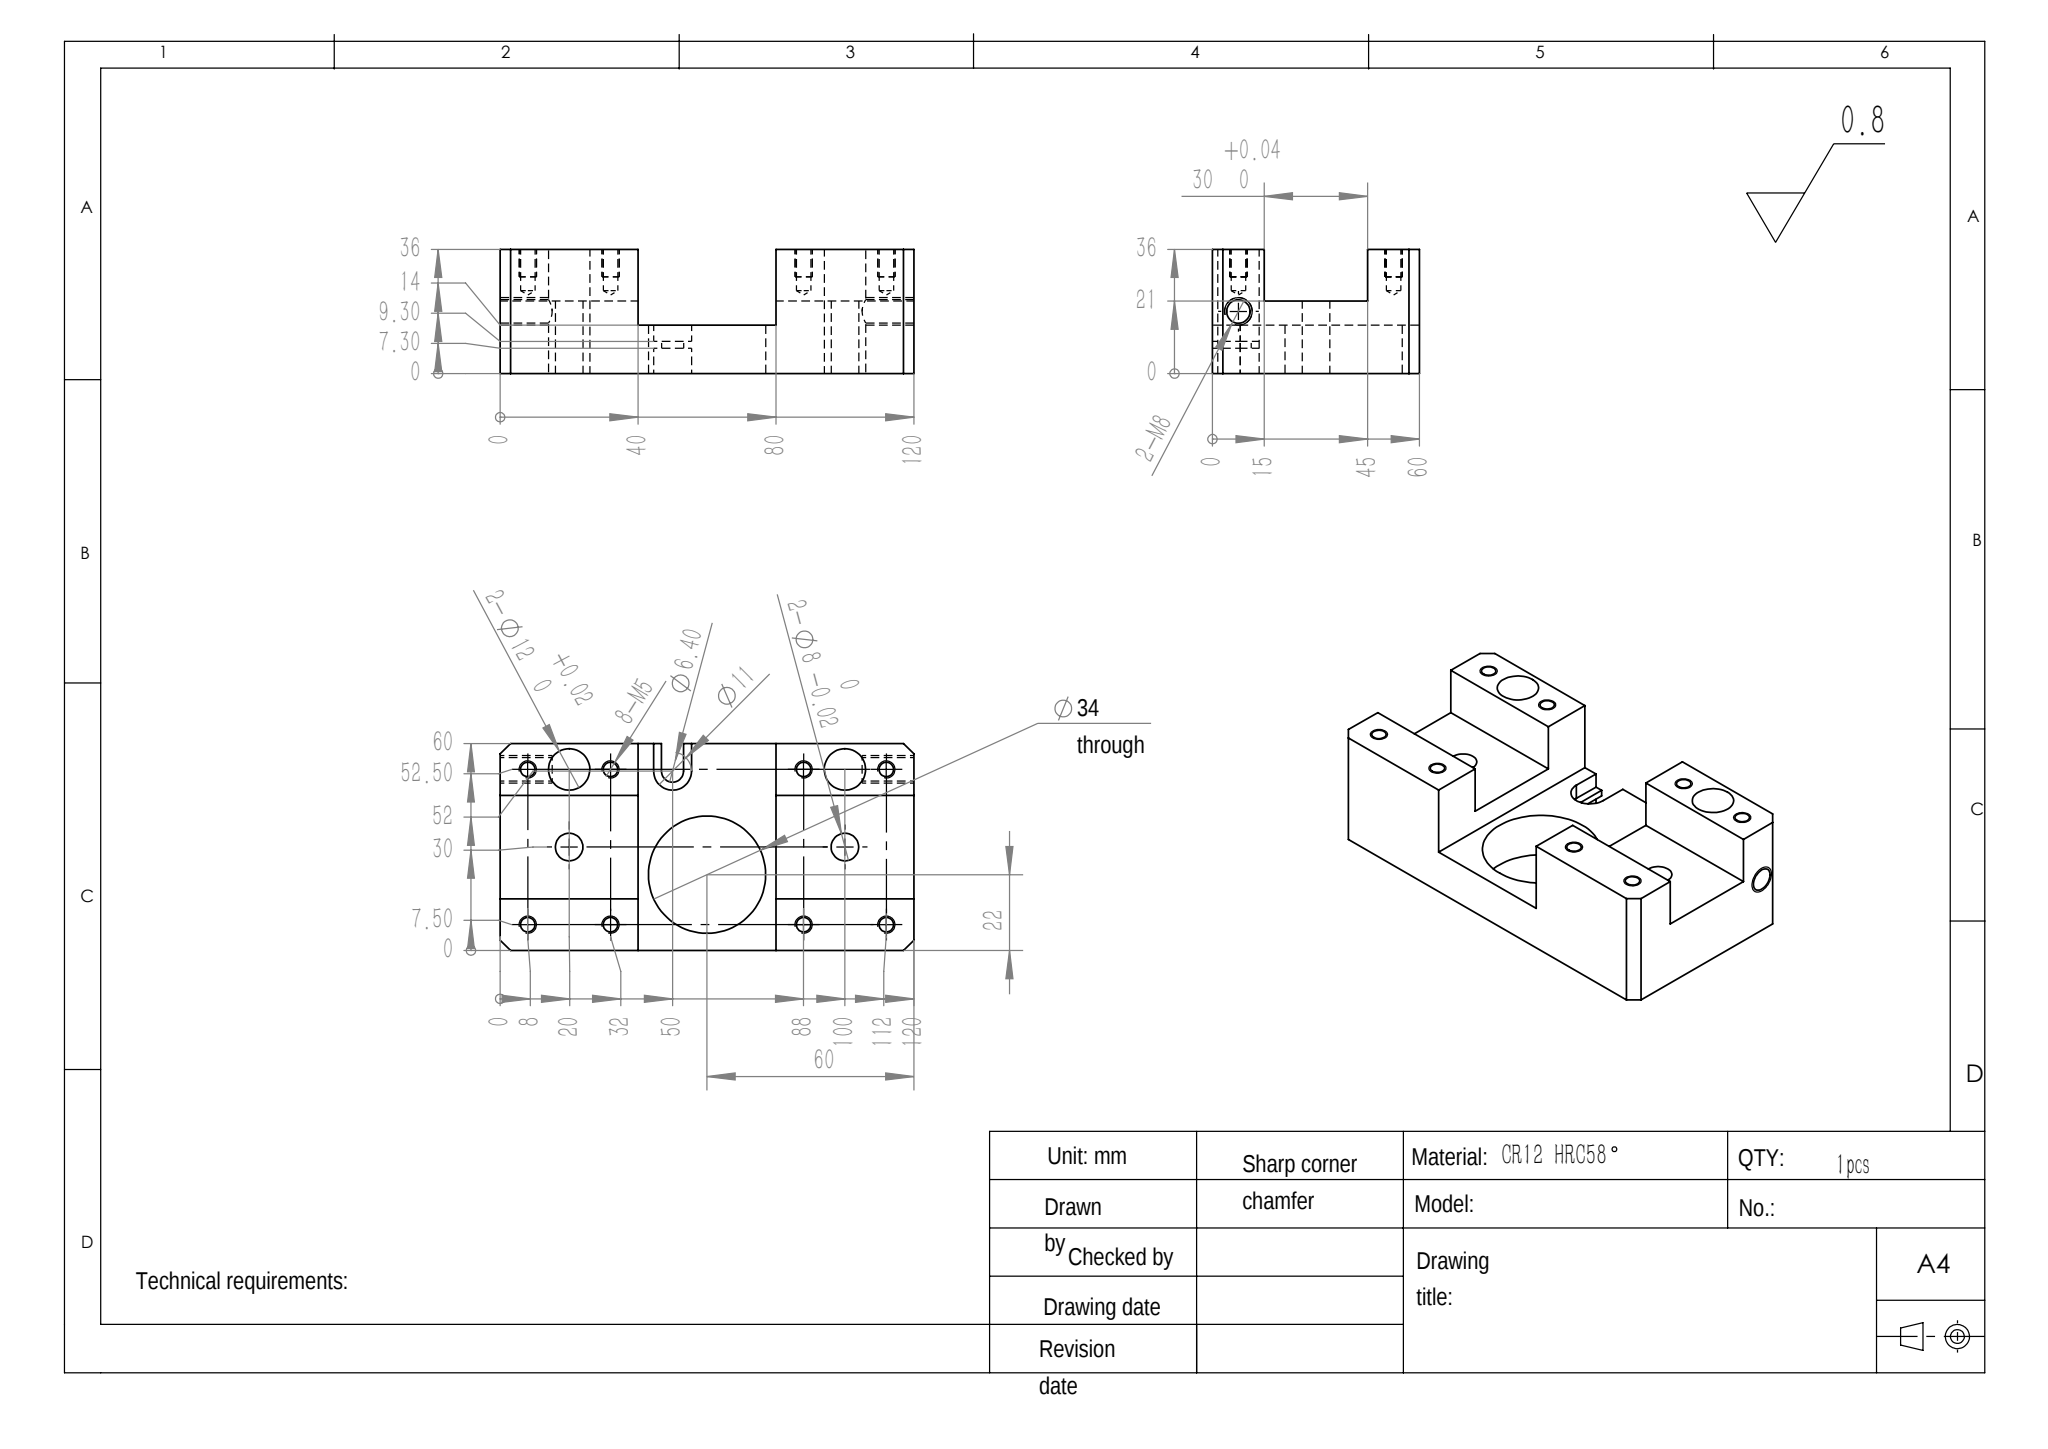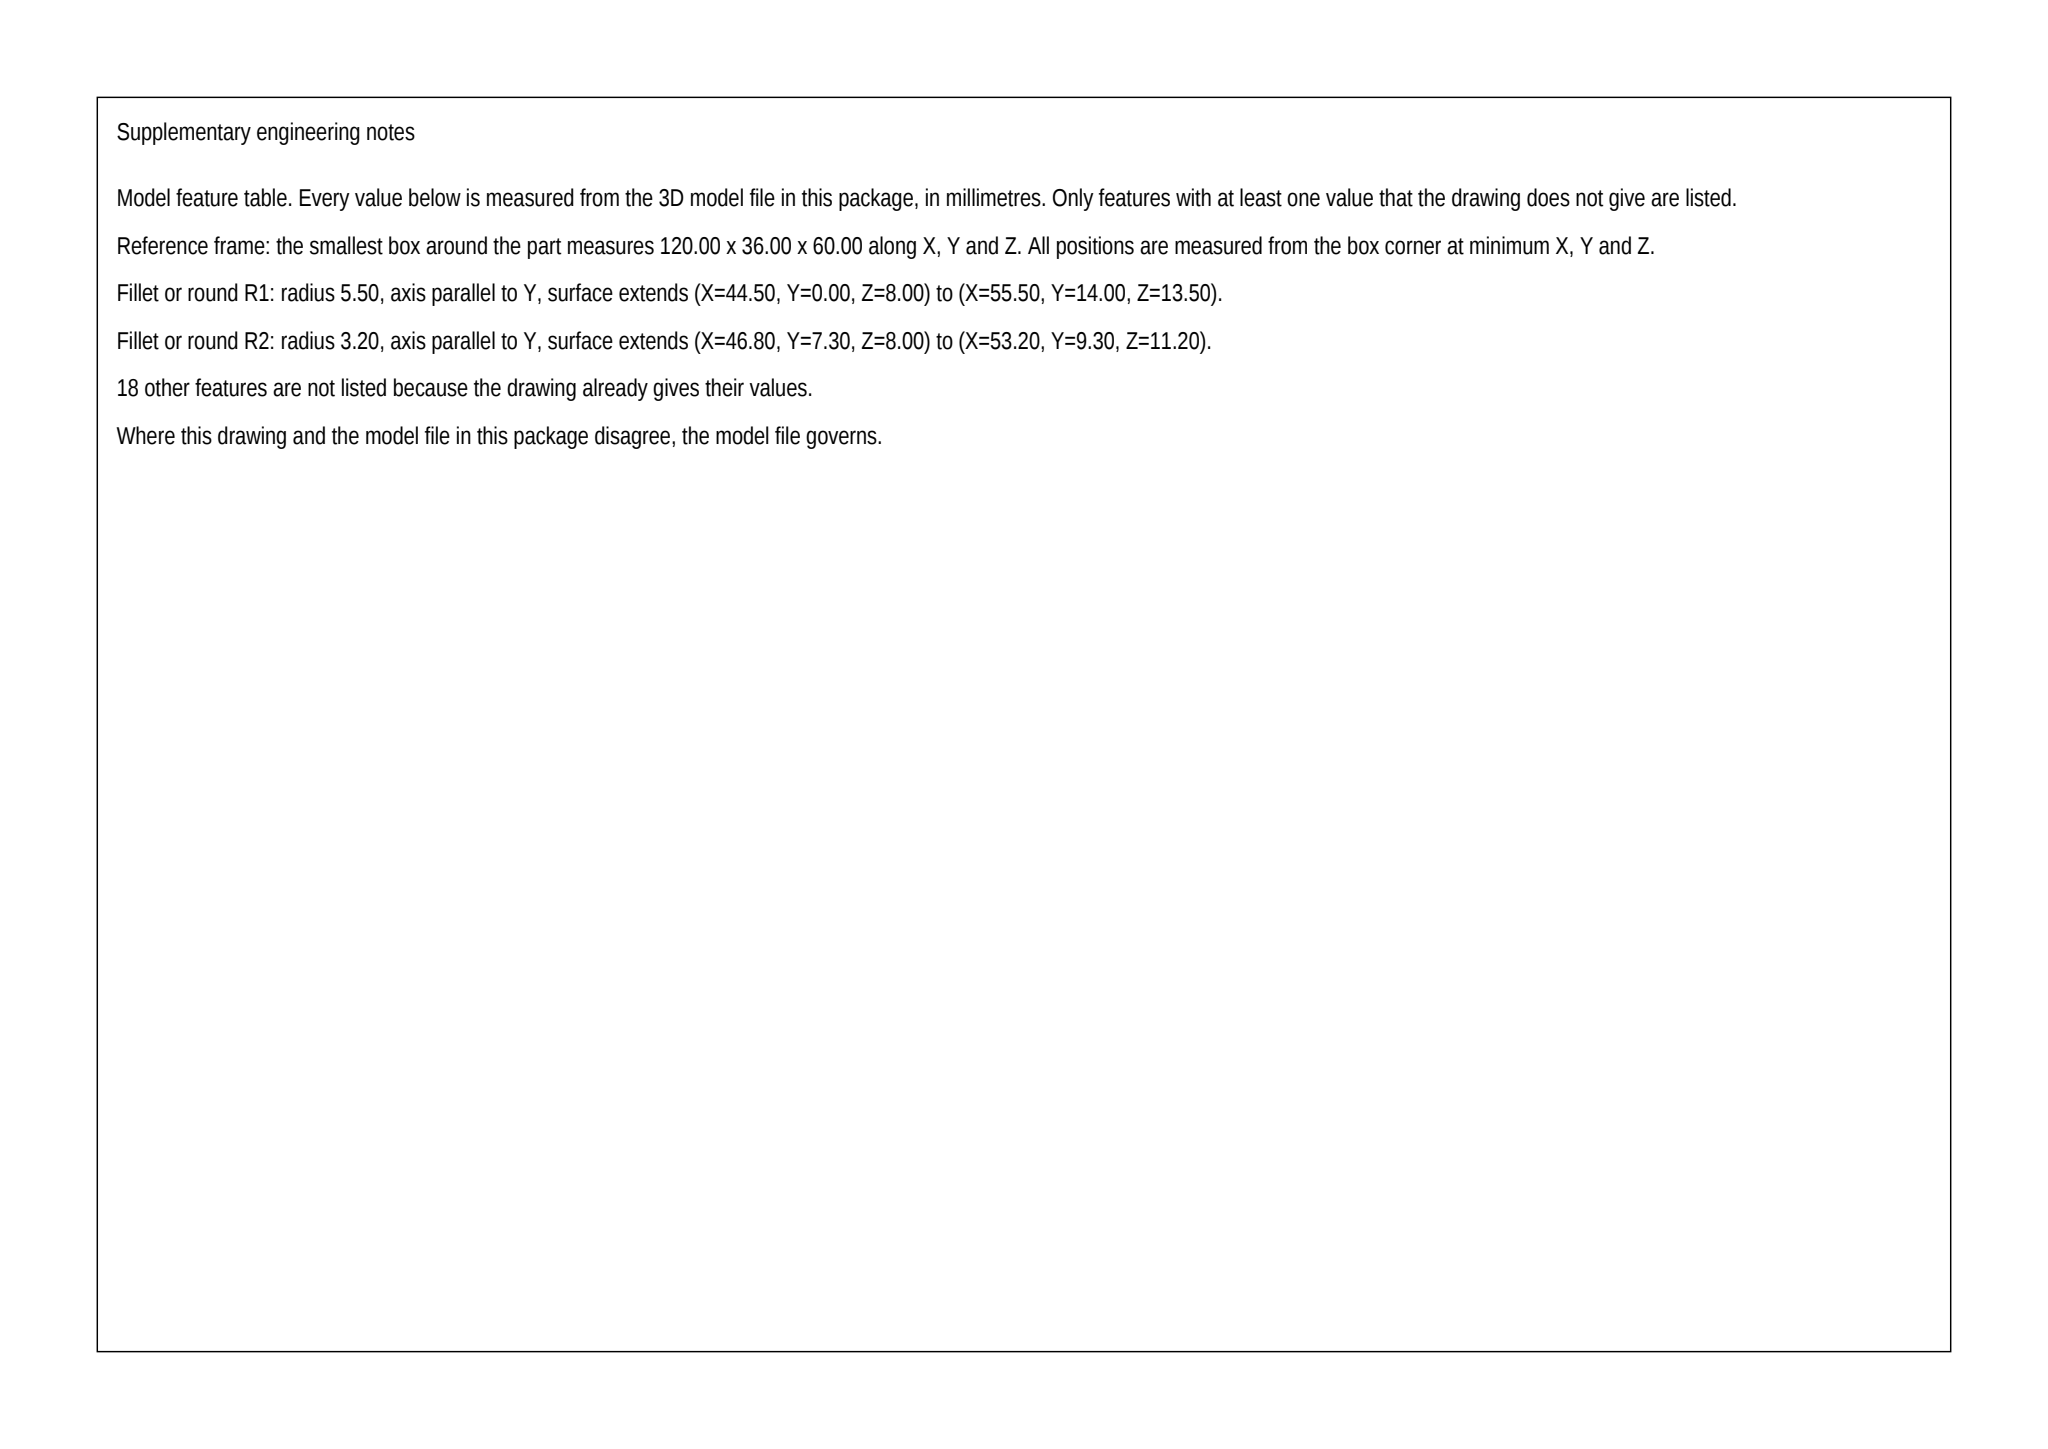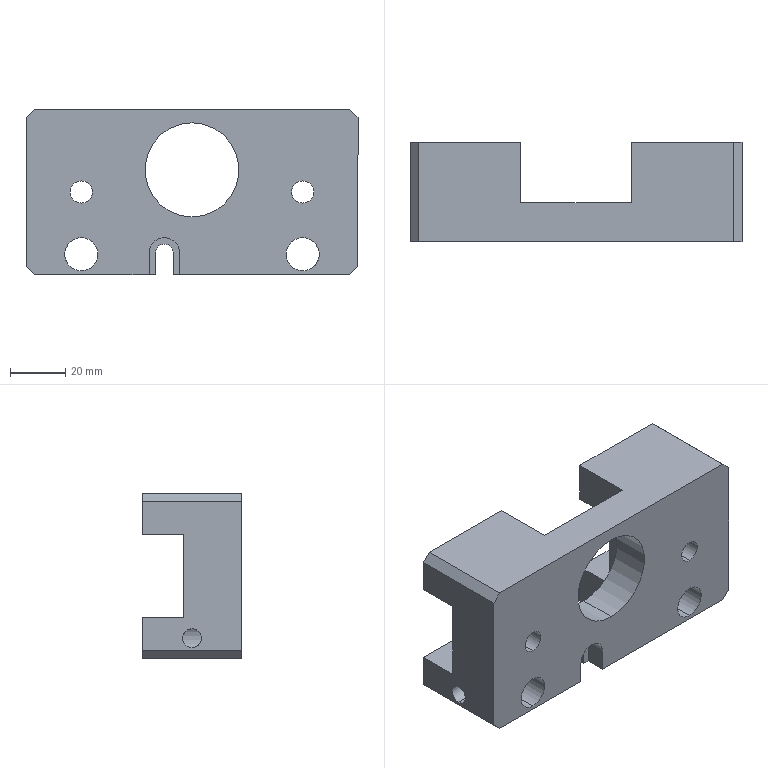Part | SolidWorks | mm | 1 solid | 83 faces | box 120 x 36 x 60 mm | volume 142614 mm3 | cylinder 36 | plane 31 | cone 16 | commonest cylinder face diameters 4.2 x16 8 x4 6.8 x4 11 x4 12 x4 34 x2 6.4 x2
build123d program:
from build123d import *

# Parameters (mm, degrees)
SKETCH1_W                                            = 120
SKETCH1_H                                            = 60
BOSS_EXTRUDE1_DEPTH                                  = 36
SKETCH2_W                                            = 87.259
SKETCH2_H                                            = 30
CUT_EXTRUDE1_DEPTH                                   = 15
M5_TAPPED_HOLE1_D                                    = 4.2
M5_TAPPED_HOLE1_DEPTH                                = 12
M5_TAPPED_HOLE1_TIP                                  = 1.262
F_12_0_12_DIAMETER_HOLE1_D                           = 12
SKETCH9_W                                            = 62.06
SKETCH9_H                                            = 30
CUT_EXTRUDE2_DEPTH                                   = 15
SKETCH10_W                                           = 40
SKETCH10_H                                           = 60
CUT_EXTRUDE3_DEPTH                                   = 22
CHAMFER1_SIZE                                        = 3
SKETCH11_R                                           = 4
BOSS_EXTRUDE2_DEPTH                                  = 6
SKETCH12_R                                           = 4
BOSS_EXTRUDE3_DEPTH                                  = 6
HOLE_SIZE_ACCORDING_TO_HEXALOBULAR_SOCKE_D           = 6.4
HOLE_SIZE_ACCORDING_TO_HEXALOBULAR_SOCKE_CBORE_D     = 11
HOLE_SIZE_ACCORDING_TO_HEXALOBULAR_SOCKE_CBORE_DEPTH = 4.7
CUT_EXTRUDE4_START                                   = -2
SKETCH15_R                                           = 5.5
CUT_EXTRUDE4_DEPTH                                   = 10
SKETCH16_W                                           = 11
SKETCH16_H                                           = 8
CUT_EXTRUDE5_DEPTH                                   = 4.7
SKETCH17_W                                           = 6.4
SKETCH17_H                                           = 8
CUT_EXTRUDE6_DEPTH                                   = 10
SKETCH18_W                                           = 11
SKETCH18_H                                           = 8
CUT_EXTRUDE7_DEPTH                                   = 26
M8_TAPPED_HOLE2_D                                    = 6.8
M8_TAPPED_HOLE2_DEPTH                                = 19.75
M8_TAPPED_HOLE2_TIP                                  = 2.043
M8_TAPPED_HOLE1_D                                    = 6.8
M8_TAPPED_HOLE1_DEPTH                                = 19.75
M8_TAPPED_HOLE1_TIP                                  = 2.043
SKETCH23_R                                           = 4
CUT_EXTRUDE8_DEPTH                                   = 137.854
SKETCH24_R                                           = 17
CUT_EXTRUDE9_DEPTH                                   = 136.956


with BuildPart() as part:
    # Sketch1 → Boss-Extrude1 (new body)
    with BuildSketch(Plane(origin=(0, 0, 0), x_dir=(1, 0, 0), z_dir=(0, 1, 0))):
        with Locations((-60, -30)):
            Rectangle(SKETCH1_W, SKETCH1_H)
    extrude(amount=BOSS_EXTRUDE1_DEPTH)

    # Sketch2 → Cut-Extrude1 (cut)
    with BuildSketch(Plane(origin=(0, 36, 0), x_dir=(1, 0, 0), z_dir=(0, 1, 0))):
        with Locations((-16.37, -30)):
            Rectangle(SKETCH2_W, SKETCH2_H)
    extrude(amount=-CUT_EXTRUDE1_DEPTH, mode=Mode.SUBTRACT)

    # M5 Tapped Hole1
    with Locations(Plane(origin=(0, 36, 0), x_dir=(-1, 0, 0), z_dir=(0, 1, 0))):
        with Locations((112, 7.5), (8, 7.5), (8, 52.5), (112, 52.5), (88, 7.5), (88, 52.5), (32, 52.5), (32, 7.5)):
            Hole(M5_TAPPED_HOLE1_D / 2, depth=M5_TAPPED_HOLE1_DEPTH)
            with Locations((0, 0, -(M5_TAPPED_HOLE1_DEPTH + M5_TAPPED_HOLE1_TIP / 2))):  # 118° drill point
                Cone(0, M5_TAPPED_HOLE1_D / 2, M5_TAPPED_HOLE1_TIP, mode=Mode.SUBTRACT)

    # 12.0 _12_ Diameter Hole1 (through all)
    with Locations(Plane.XZ):
        with Locations((-100, 7.5), (-20, 7.5)):
            Hole(F_12_0_12_DIAMETER_HOLE1_D / 2)

    # Sketch9 → Cut-Extrude2 (cut)
    with BuildSketch(Plane(origin=(0, 36, 0), x_dir=(1, 0, 0), z_dir=(0, 1, 0))):
        with Locations((-91.03, -30)):
            Rectangle(SKETCH9_W, SKETCH9_H)
    extrude(amount=-CUT_EXTRUDE2_DEPTH, mode=Mode.SUBTRACT)

    # Sketch10 → Cut-Extrude3 (cut)
    with BuildSketch(Plane(origin=(0, 36, 0), x_dir=(1, 0, 0), z_dir=(0, 1, 0))):
        with Locations((-60, -30)):
            Rectangle(SKETCH10_W, SKETCH10_H)
    extrude(amount=-CUT_EXTRUDE3_DEPTH, mode=Mode.SUBTRACT)

    # Chamfer1
    chamfer1_edges = [part.edges().sort_by_distance(p)[0] for p in [
        (-120, 18, 0),
        (0, 18, 0),
        (0, 18, 60),
        (-120, 18, 60),
    ]]
    chamfer(chamfer1_edges, length=CHAMFER1_SIZE)

    # Sketch11 → Boss-Extrude2 (add)
    with BuildSketch(Plane(origin=(0, 21, 0), x_dir=(1, 0, 0), z_dir=(0, 1, 0))):
        with Locations(Location((-20, -30, 0), (0, 0, 270))):
            Circle(SKETCH11_R)
    extrude(amount=BOSS_EXTRUDE2_DEPTH)

    # Sketch12 → Boss-Extrude3 (add)
    with BuildSketch(Plane(origin=(0, 21, 0), x_dir=(1, 0, 0), z_dir=(0, 1, 0))):
        with Locations(Location((-100, -30, 0), (0, 0, 270))):
            Circle(SKETCH12_R)
    extrude(amount=BOSS_EXTRUDE3_DEPTH)

    # Hole Size according to Hexalobular Socke (through all)
    with Locations(Plane(origin=(0, 14, 0), x_dir=(-1, 0, 0), z_dir=(0, 1, 0))):
        with Locations((70, 8)):
            CounterBoreHole(HOLE_SIZE_ACCORDING_TO_HEXALOBULAR_SOCKE_D / 2, HOLE_SIZE_ACCORDING_TO_HEXALOBULAR_SOCKE_CBORE_D / 2, HOLE_SIZE_ACCORDING_TO_HEXALOBULAR_SOCKE_CBORE_DEPTH)

    # Sketch15 → Cut-Extrude4 (cut)
    with BuildSketch(Plane(origin=(0, 9.3, 0), x_dir=(1, 0, 0), z_dir=(0, 1, 0)).offset(CUT_EXTRUDE4_START)):
        with Locations(Location((-70, -8, 0), (0, 0, 270))):
            Circle(SKETCH15_R)
    extrude(amount=-CUT_EXTRUDE4_DEPTH, mode=Mode.SUBTRACT)

    # Sketch16 → Cut-Extrude5 (cut)
    with BuildSketch(Plane(origin=(0, 14, 0), x_dir=(1, 0, 0), z_dir=(0, 1, 0))):
        with Locations((-70, -4)):
            Rectangle(SKETCH16_W, SKETCH16_H)
    extrude(amount=-CUT_EXTRUDE5_DEPTH, mode=Mode.SUBTRACT)

    # Sketch17 → Cut-Extrude6 (cut)
    with BuildSketch(Plane(origin=(0, 9.3, 0), x_dir=(1, 0, 0), z_dir=(0, 1, 0))):
        with Locations((-70, -4)):
            Rectangle(SKETCH17_W, SKETCH17_H)
    extrude(amount=-CUT_EXTRUDE6_DEPTH, mode=Mode.SUBTRACT)

    # Sketch18 → Cut-Extrude7 (cut)
    with BuildSketch(Plane.XZ.offset(-7.3)):
        with Locations((-70, 4)):
            Rectangle(SKETCH18_W, SKETCH18_H)
    extrude(amount=CUT_EXTRUDE7_DEPTH, mode=Mode.SUBTRACT)

    # M8 Tapped Hole2
    with Locations(Plane.ZY.offset(120)):
        with Locations((7.5, 18)):
            Hole(M8_TAPPED_HOLE2_D / 2, depth=M8_TAPPED_HOLE2_DEPTH)
            with Locations((0, 0, -(M8_TAPPED_HOLE2_DEPTH + M8_TAPPED_HOLE2_TIP / 2))):  # 118° drill point
                Cone(0, M8_TAPPED_HOLE2_D / 2, M8_TAPPED_HOLE2_TIP, mode=Mode.SUBTRACT)

    # M8 Tapped Hole1
    with Locations(Plane(origin=(0, 0, 0), x_dir=(0, 0, -1), z_dir=(1, 0, 0))):
        with Locations((-7.5, 18)):
            Hole(M8_TAPPED_HOLE1_D / 2, depth=M8_TAPPED_HOLE1_DEPTH)
            with Locations((0, 0, -(M8_TAPPED_HOLE1_DEPTH + M8_TAPPED_HOLE1_TIP / 2))):  # 118° drill point
                Cone(0, M8_TAPPED_HOLE1_D / 2, M8_TAPPED_HOLE1_TIP, mode=Mode.SUBTRACT)

    # Sketch23 → Cut-Extrude8 (cut, through all)
    with BuildSketch(Plane(origin=(0, 27, 0), x_dir=(1, 0, 0), z_dir=(0, 1, 0))):
        with Locations(Location((-20, -30, 0), (0, 0, 270))):
            Circle(SKETCH23_R)
        with Locations(Location((-100, -30, 0), (0, 0, 270))):
            Circle(SKETCH23_R)
    extrude(amount=-CUT_EXTRUDE8_DEPTH, mode=Mode.SUBTRACT)

    # Sketch24 → Cut-Extrude9 (cut, through all)
    with BuildSketch(Plane(origin=(0, 14, 0), x_dir=(1, 0, 0), z_dir=(0, 1, 0))):
        with Locations(Location((-60, -38, 0), (0, 0, 270))):
            Circle(SKETCH24_R)
    extrude(amount=-CUT_EXTRUDE9_DEPTH, mode=Mode.SUBTRACT)


solid = part.part